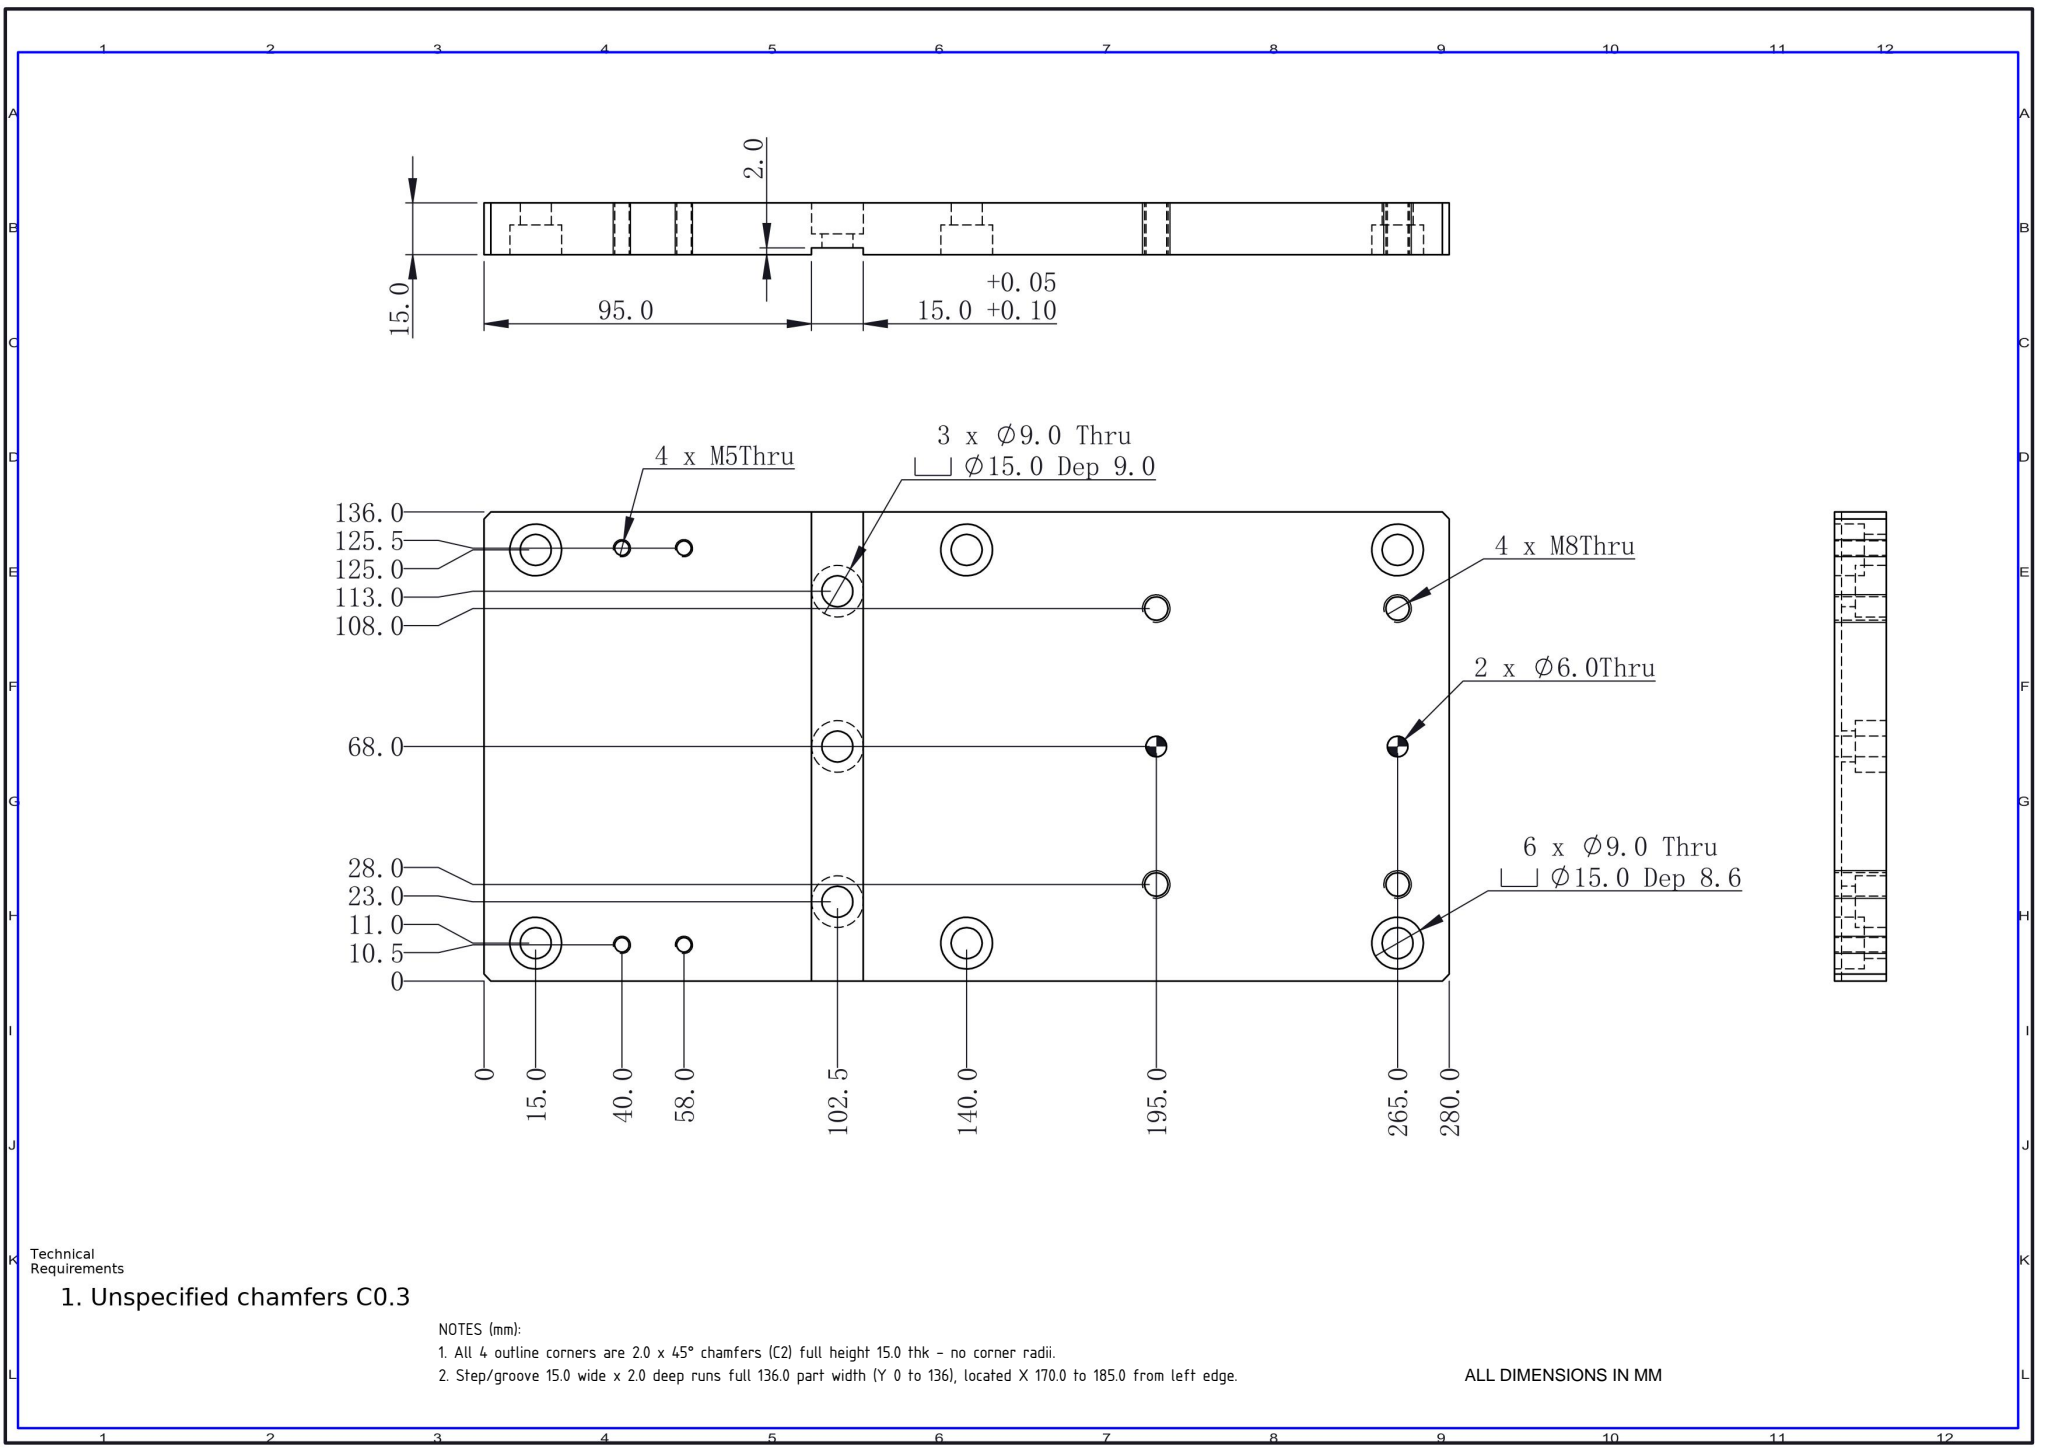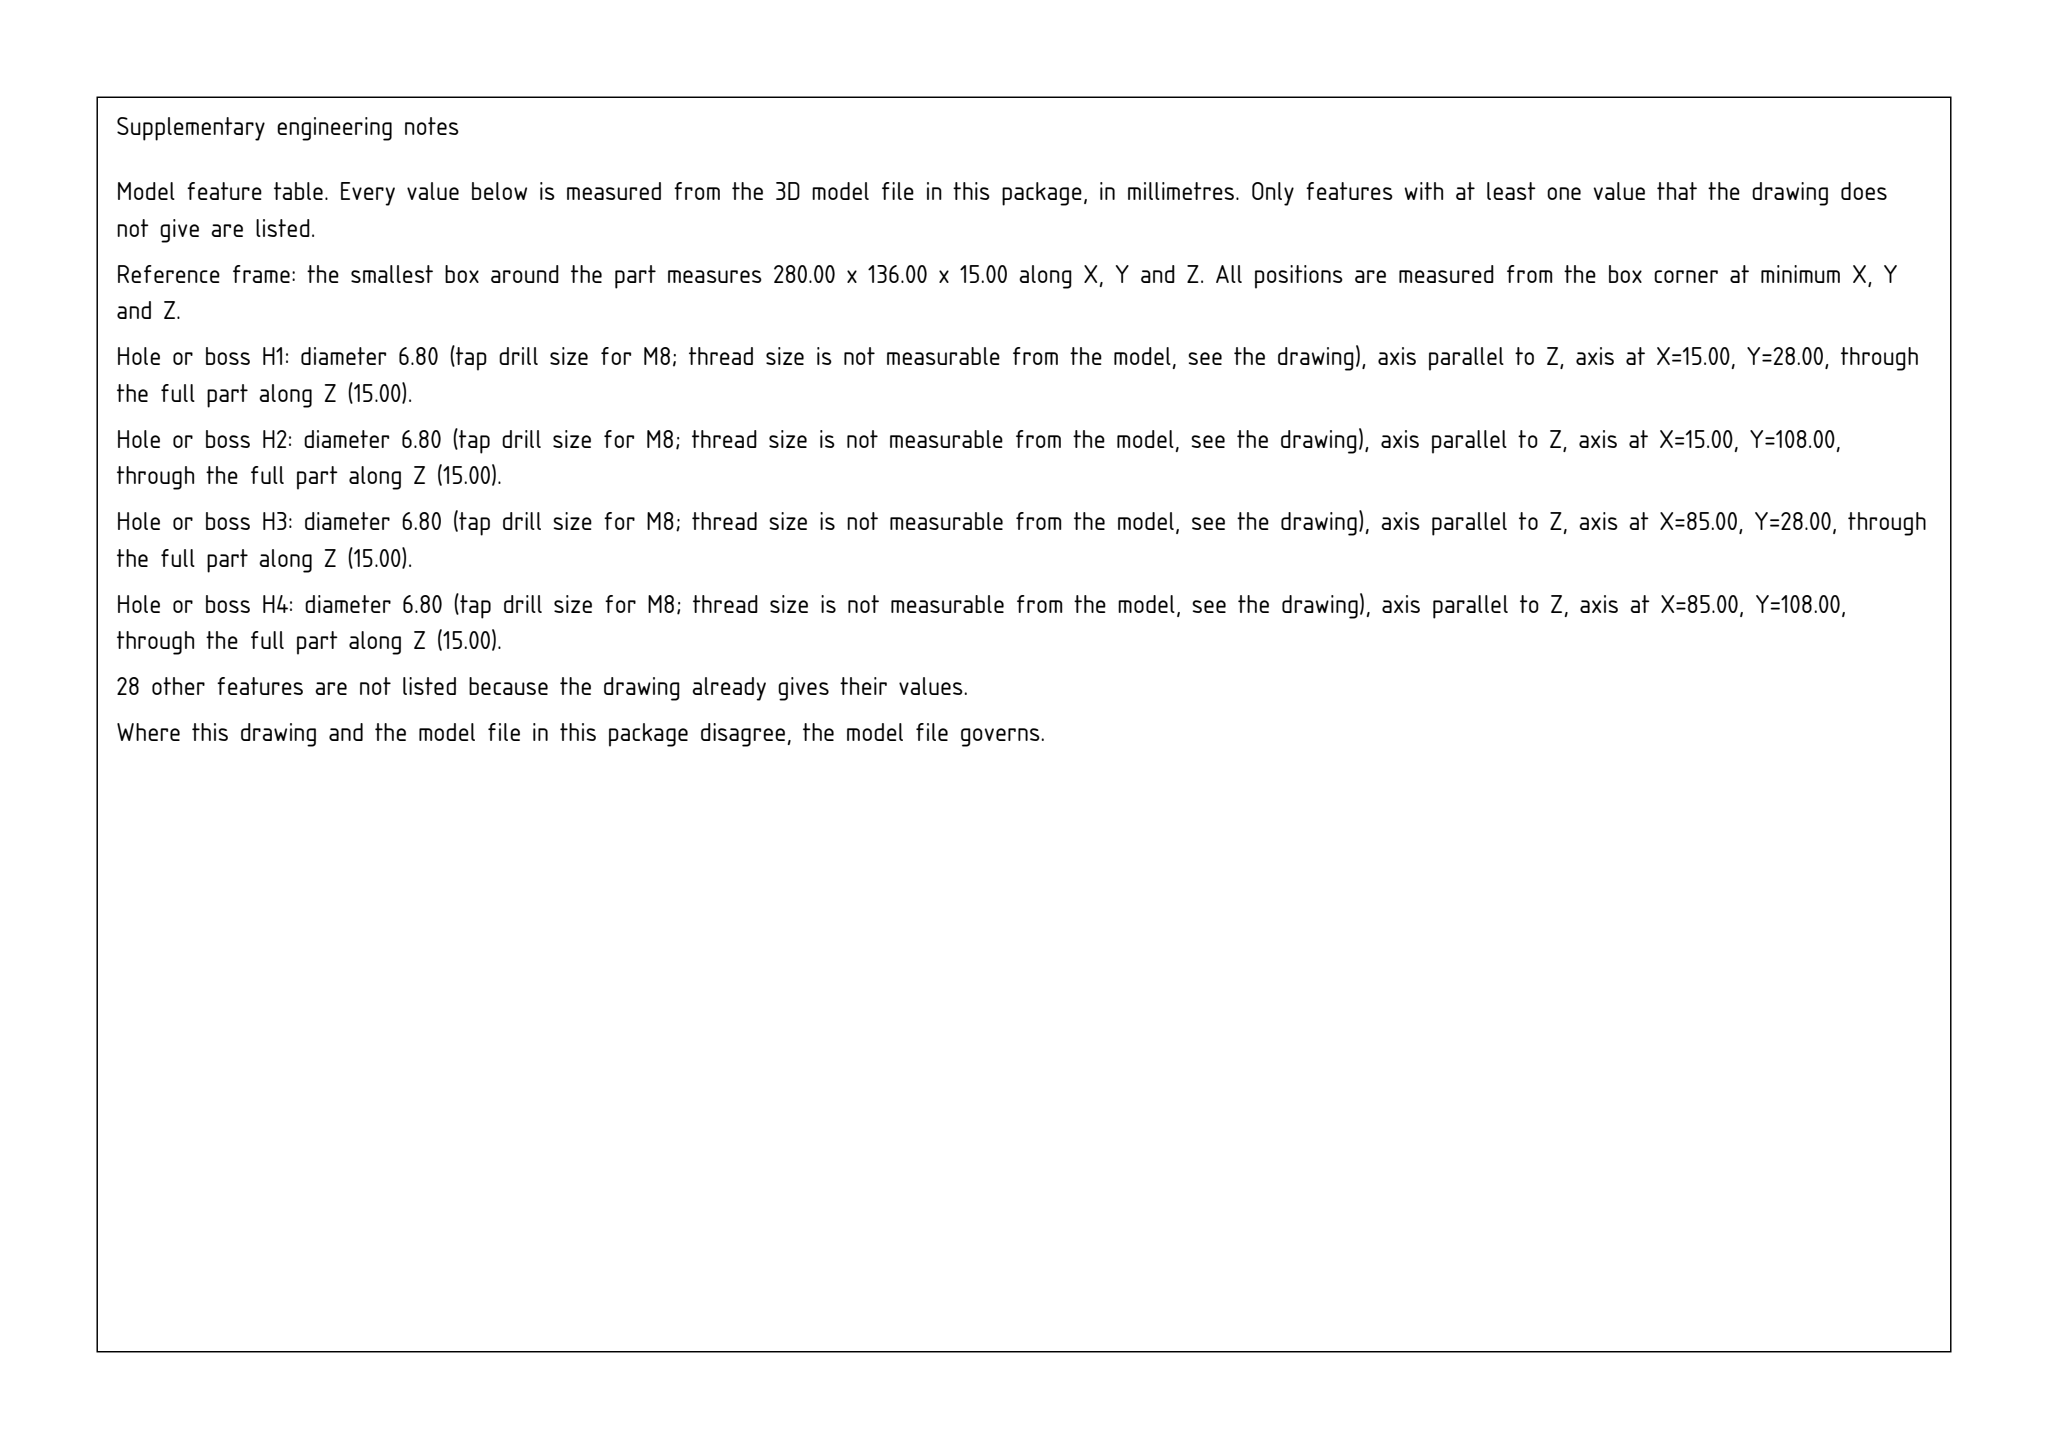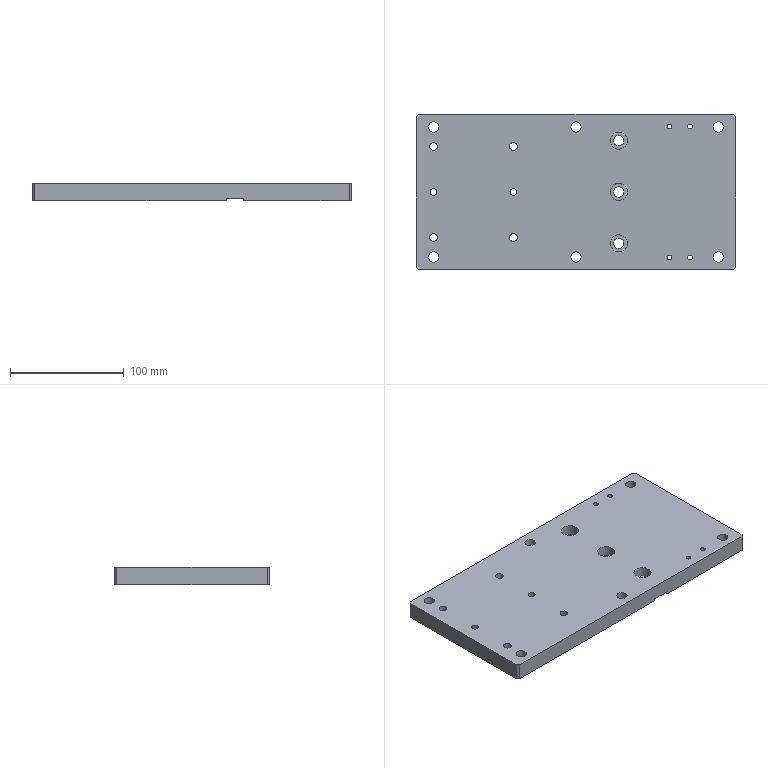Part | SolidWorks | mm | 1 solid | 79 faces | box 280 x 136 x 15 mm | volume 546045 mm3 | cylinder 56 | plane 23 | commonest cylinder face diameters 15 x18 9 x18 6.8 x8 4.2 x8 6 x4
Drawing notes:
All 4 outline corners are 2.0 x 45° chamfers (C2) full height 15.0 thk - no corner radii. | from the solid: inclined_planes: 4 faces at 45°/45°/90°, size [2.0, 2.0, 15.0] at corners [0,0,0], [0,134,0], [278,0,0], [278,134,0]
Step/groove 15.0 wide x 2.0 deep runs full 136.0 part width (Y 0 to 136), located X 170.0 to 185.0 from left edge. | from the solid: axis_planes: x=170.0 and x=185.0 faces extent y [0,136] z [0,2]; z=2.0 face extent x [170,185], y [0,136]
build123d program:
from build123d import *

# Parameters (mm, degrees)
SKETCH1_W                                       = 280
SKETCH1_H                                       = 136
BOSS_EXTRUDE1_DEPTH                             = 15
SKETCH2_W                                       = 15
SKETCH2_H                                       = 136
CUT_EXTRUDE1_DEPTH                              = 2
M5_TAPPED_HOLE1_D                               = 4.2
M8_HEX_SOCKET_HEAD_CAP_SCREW_CBORE2_D           = 9
M8_HEX_SOCKET_HEAD_CAP_SCREW_CBORE2_CBORE_D     = 15
M8_HEX_SOCKET_HEAD_CAP_SCREW_CBORE2_CBORE_DEPTH = 8.6
CHAMFER1_SIZE                                   = 2
M8_HEX_SOCKET_HEAD_CAP_SCREW_CBORE4_D           = 9
M8_HEX_SOCKET_HEAD_CAP_SCREW_CBORE4_CBORE_D     = 15
M8_HEX_SOCKET_HEAD_CAP_SCREW_CBORE4_CBORE_DEPTH = 9
M8_TAPPED_HOLE1_D                               = 6.8
SIZE_MM_DOWEL_PIN_HOLE0_D                       = 6


with BuildPart() as part:
    # Sketch1 → Boss-Extrude1 (new body)
    with BuildSketch(Plane.XY):
        with Locations((140, 68)):
            Rectangle(SKETCH1_W, SKETCH1_H)
    extrude(amount=BOSS_EXTRUDE1_DEPTH)

    # Sketch2 → Cut-Extrude1 (cut)
    with BuildSketch(Plane(origin=(0, 0, 0), x_dir=(-1, 0, 0), z_dir=(0, 0, -1))):
        with Locations((-177.5, 68)):
            Rectangle(SKETCH2_W, SKETCH2_H)
    extrude(amount=-CUT_EXTRUDE1_DEPTH, mode=Mode.SUBTRACT)

    # M5 Tapped Hole1 (through all)
    with Locations(Plane(origin=(0, 0, 0), x_dir=(-1, 0, 0), z_dir=(0, 0, -1))):
        with Locations((-240, 125.5), (-222, 125.5), (-240, 10.5), (-222, 10.5)):
            Hole(M5_TAPPED_HOLE1_D / 2)

    # M8 Hex Socket Head Cap Screw CBORE2 (through all)
    with Locations(Plane(origin=(0, 0, 0), x_dir=(-1, 0, 0), z_dir=(0, 0, -1))):
        with Locations((-265, 11), (-140, 11), (-140, 125), (-265, 125), (-15, 11), (-15, 125)):
            CounterBoreHole(M8_HEX_SOCKET_HEAD_CAP_SCREW_CBORE2_D / 2, M8_HEX_SOCKET_HEAD_CAP_SCREW_CBORE2_CBORE_D / 2, M8_HEX_SOCKET_HEAD_CAP_SCREW_CBORE2_CBORE_DEPTH)

    # Chamfer1
    chamfer1_edges = [part.edges().sort_by_distance(p)[0] for p in [
        (0, 136, 7.5),
        (280, 136, 7.5),
        (280, 0, 7.5),
        (0, 0, 7.5),
    ]]
    chamfer(chamfer1_edges, length=CHAMFER1_SIZE)

    # M8 Hex Socket Head Cap Screw CBORE4 (through all)
    with Locations(Plane.XY.offset(15)):
        with Locations((177.5, 113), (177.5, 68), (177.5, 23)):
            CounterBoreHole(M8_HEX_SOCKET_HEAD_CAP_SCREW_CBORE4_D / 2, M8_HEX_SOCKET_HEAD_CAP_SCREW_CBORE4_CBORE_D / 2, M8_HEX_SOCKET_HEAD_CAP_SCREW_CBORE4_CBORE_DEPTH)

    # M8 Tapped Hole1 (through all)
    with Locations(Plane(origin=(0, 0, 0), x_dir=(-1, 0, 0), z_dir=(0, 0, -1))):
        with Locations((-85, 108), (-15, 108), (-15, 28), (-85, 28)):
            Hole(M8_TAPPED_HOLE1_D / 2)

    # Size mm Dowel Pin Hole0 (through all)
    with Locations(Plane(origin=(0, 0, 0), x_dir=(-1, 0, 0), z_dir=(0, 0, -1))):
        with Locations((-15, 68), (-85, 68)):
            Hole(SIZE_MM_DOWEL_PIN_HOLE0_D / 2)


solid = part.part